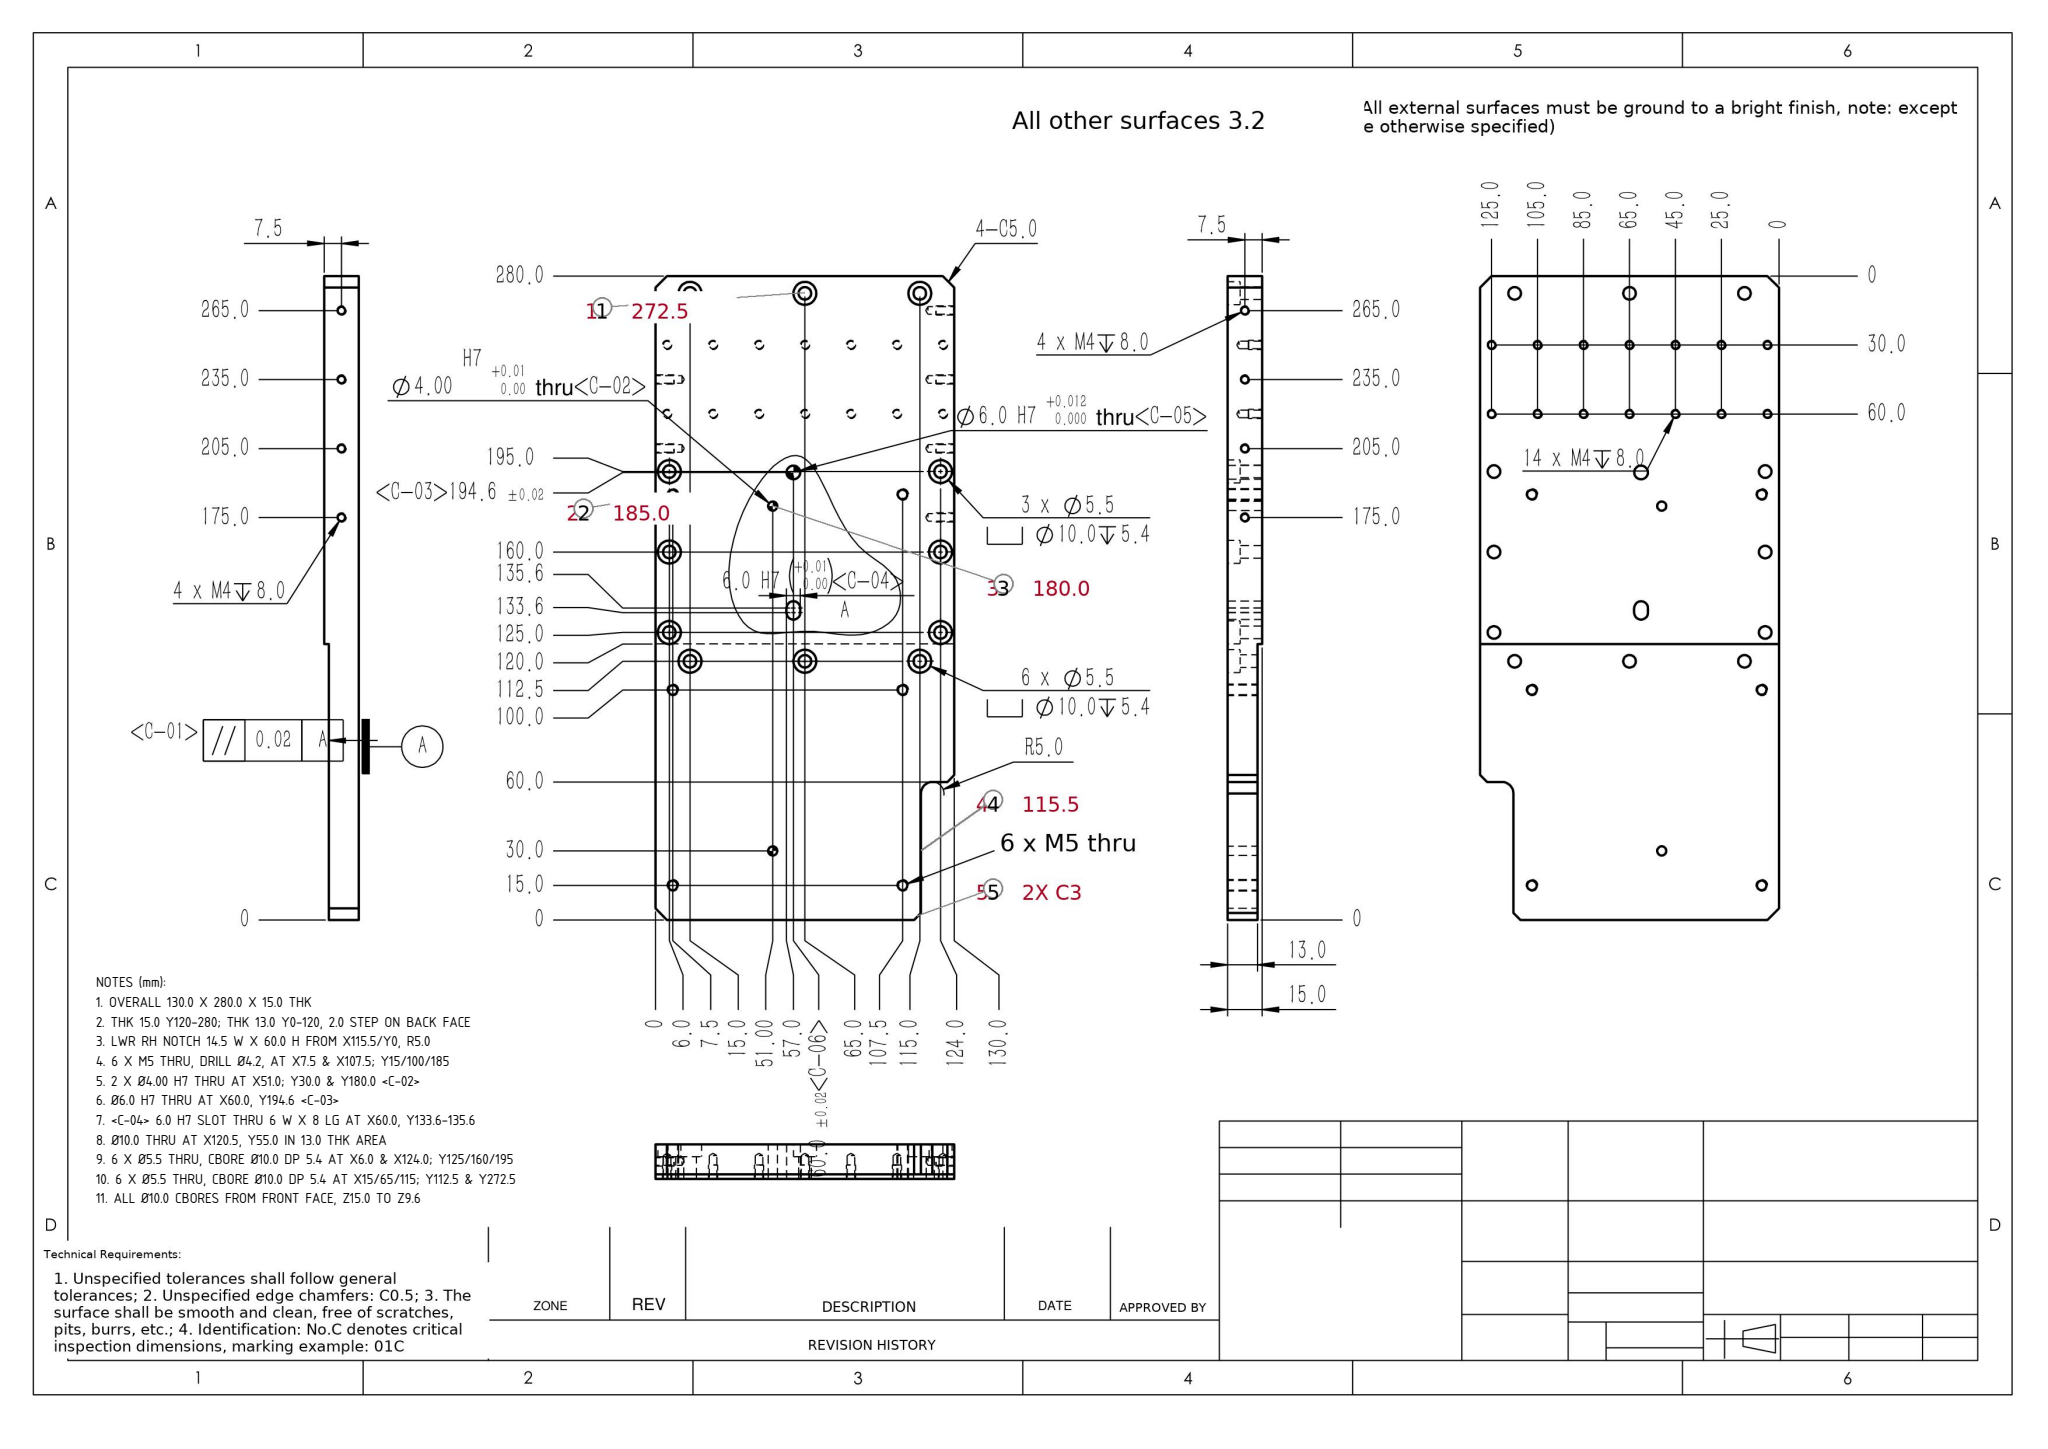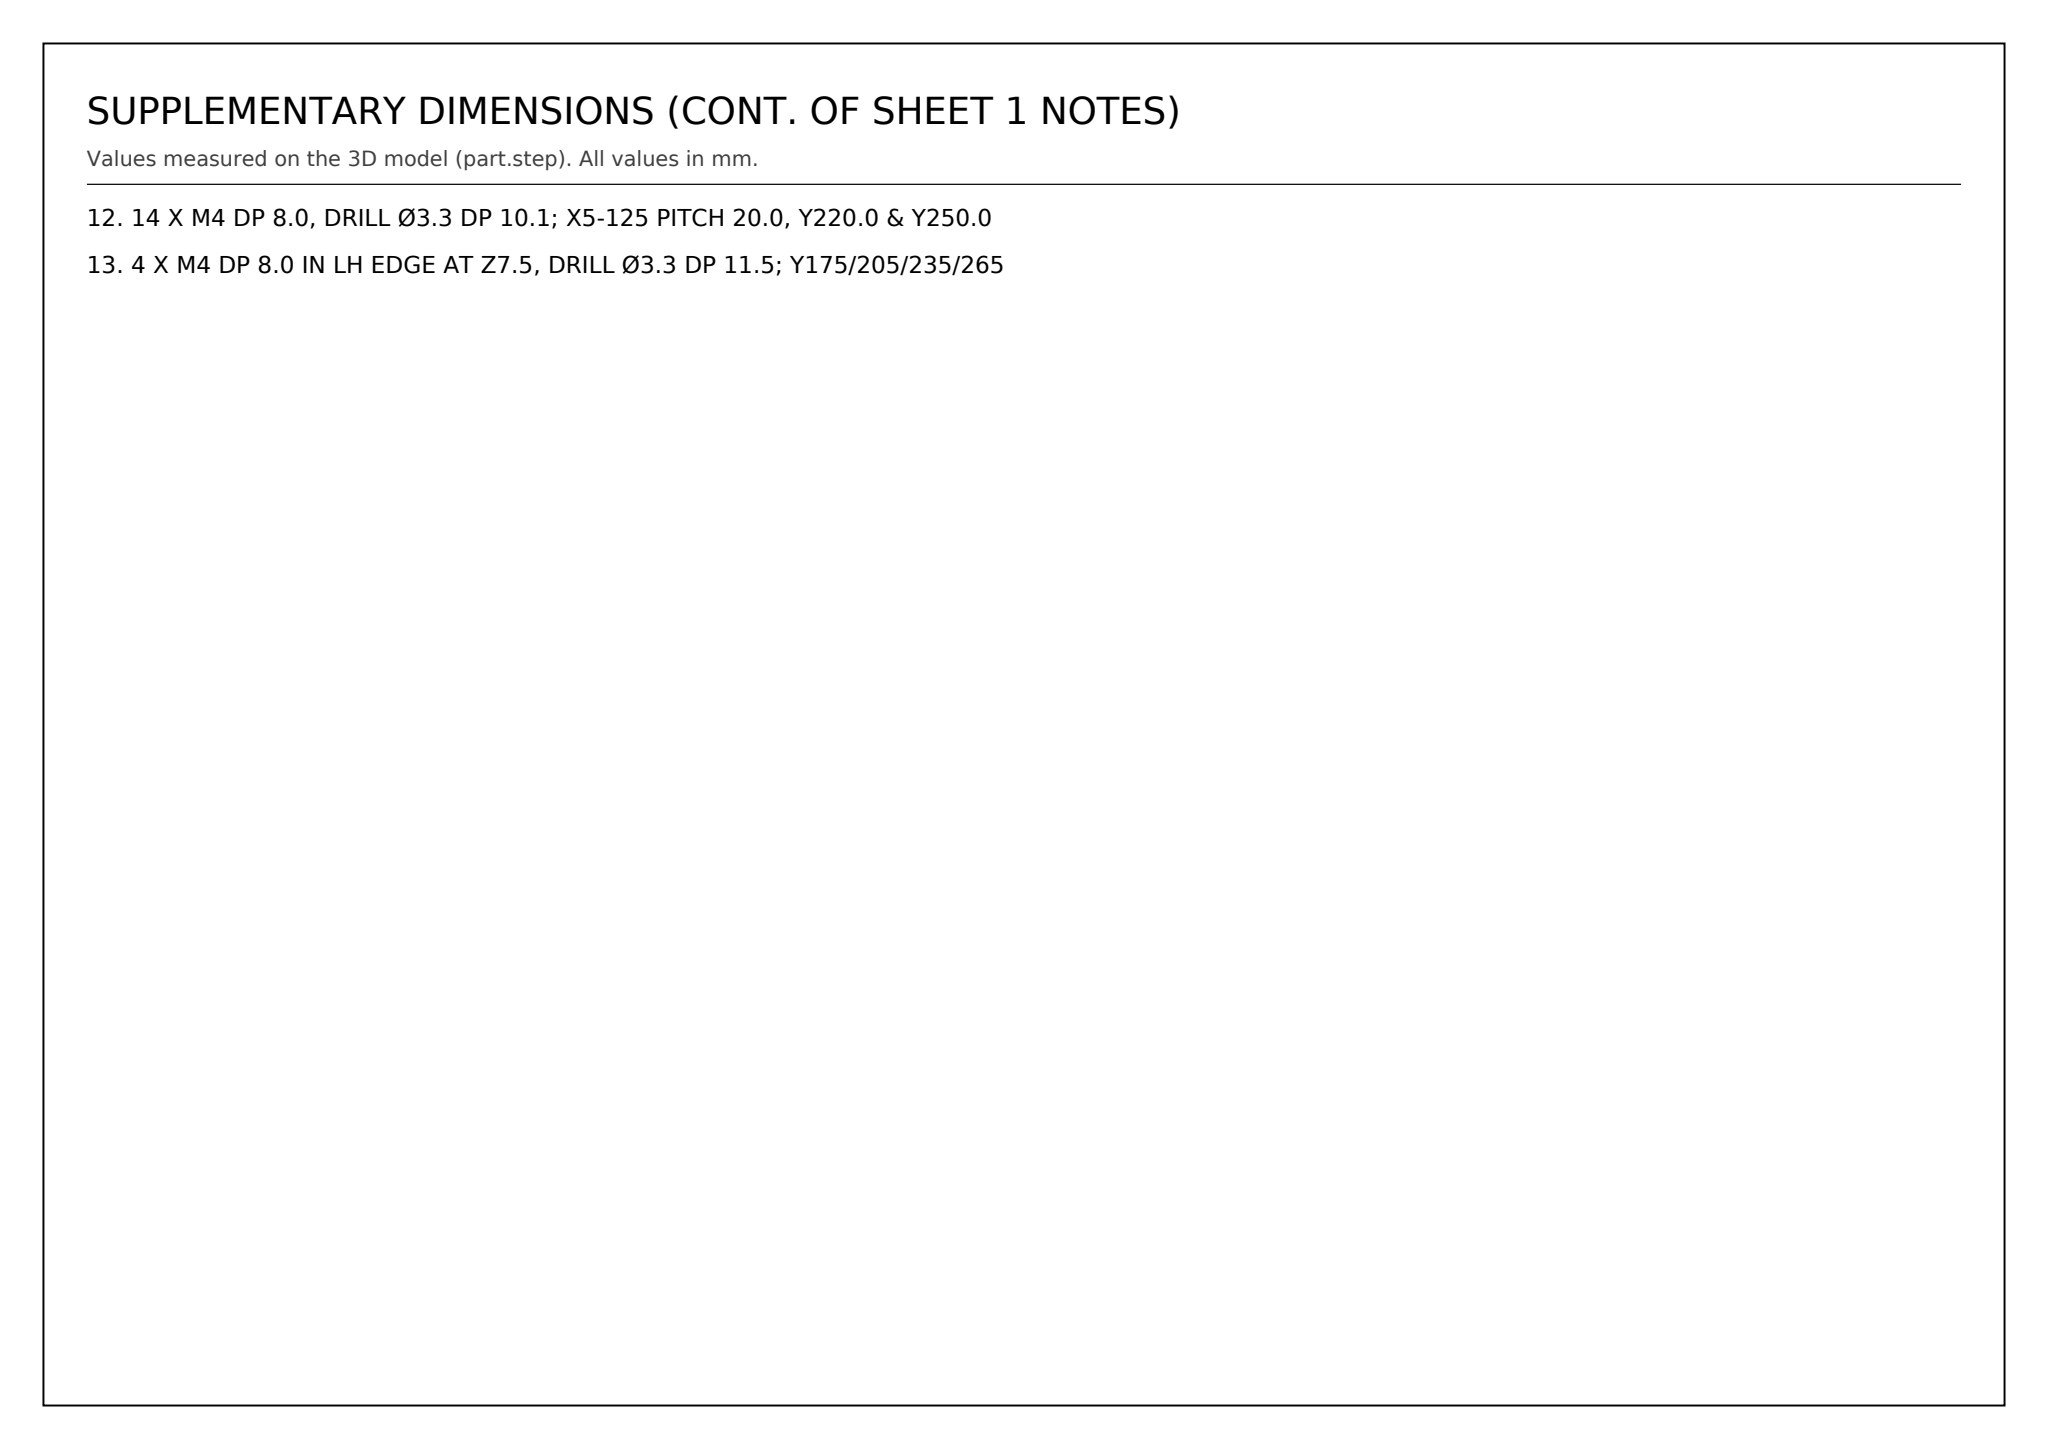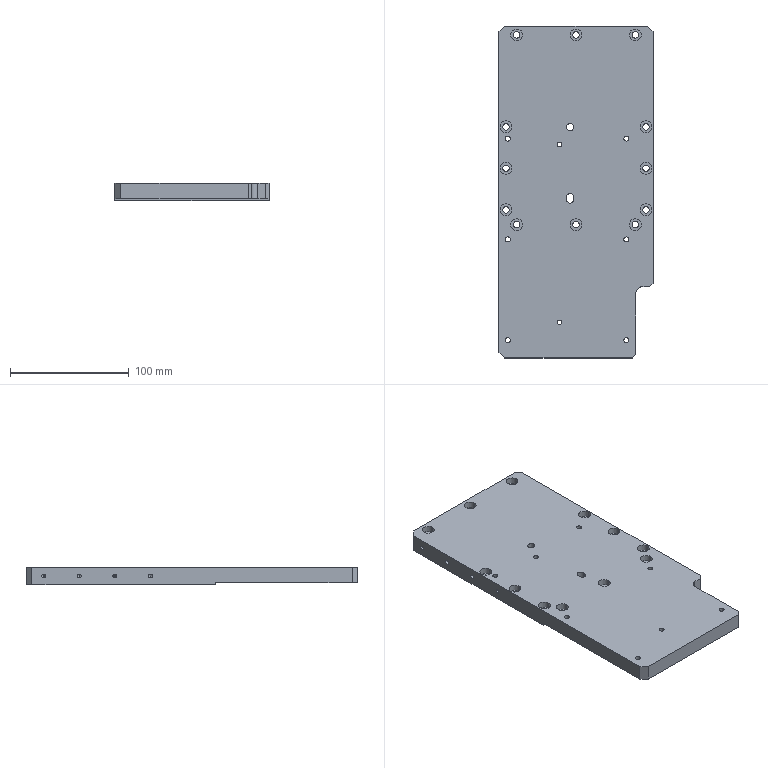Part | SolidWorks | mm | 1 solid | 186 faces | box 130 x 280 x 15 mm | volume 490647 mm3 | cylinder 113 | cone 44 | plane 29 | commonest cylinder face diameters 3.3 x44 10 x25 5.5 x24 4.2 x12 6 x4 4 x4
Drawing notes:
OVERALL 130.0 X 280.0 X 15.0 THK | from the solid: bbox_xyz [130.0, 280.0, 15.0]
THK 15.0 Y120-280; THK 13.0 Y0-120, 2.0 STEP ON BACK FACE | from the solid: z planes 0/2.0/15.0; y plane 120.0; hole len 13.0 at Y15/30/100 vs 15.0 at Y180/185
LWR RH NOTCH 14.5 W X 60.0 H FROM X115.5/Y0, R5.0 | from the solid: x plane 115.5 vs bbox x=130.0; y plane 60.0
6 X M5 THRU, DRILL Ø4.2, AT X7.5 & X107.5; Y15/100/185 | from the solid: Ø4.2 z-holes at (7.5/107.5, 15/100/185), len 13.0 & 15.0 thru
2 X Ø4.00 H7 THRU AT X51.0; Y30.0 & Y180.0 <C-02> | from the solid: Ø4.0 z-holes at (51,30) len 13.0 and (51,180) len 15.0
Ø6.0 H7 THRU AT X60.0, Y194.6 <C-03> | from the solid: Ø6.0 z-hole at (60,194.6) len 15.0
<C-04> 6.0 H7 SLOT THRU 6 W X 8 LG AT X60.0, Y133.6-135.6 | from the solid: Ø6.0 at (60,133.6) & (60,135.6) len 15.0; x planes 57.0 & 63.0
Ø10.0 THRU AT X120.5, Y55.0 IN 13.0 THK AREA | from the solid: Ø10.0 cyl at (120.5,55.0) len 13.0
6 X Ø5.5 THRU, CBORE Ø10.0 DP 5.4 AT X6.0 & X124.0; Y125/160/195 | from the solid: Ø5.5/Ø10.0 at (6,125)(6,160)(6,195)(124,125)(124,160)(124,195)
6 X Ø5.5 THRU, CBORE Ø10.0 DP 5.4 AT X15/65/115; Y112.5 & Y272.5 | from the solid: Ø5.5/Ø10.0 at (15/65/115, 112.5) and (15/65/115, 272.5)
ALL Ø10.0 CBORES FROM FRONT FACE, Z15.0 TO Z9.6 | from the solid: Ø10.0 cyl len 5.4 x12; z plane 9.6 count 12
14 X M4 DP 8.0, DRILL Ø3.3 DP 10.1; X5-125 PITCH 20.0, Y220.0 & Y250.0 | from the solid: Ø3.3 z-axis len 10.1 at x=5,25,45,65,85,105,125; y=220,250
4 X M4 DP 8.0 IN LH EDGE AT Z7.5, DRILL Ø3.3 DP 11.5; Y175/205/235/265 | from the solid: Ø3.3 x-axis len 11.5 at y=175,205,235,265, z=7.5
build123d program:
from build123d import *

# Parameters (mm, degrees)
SKETCH1_W                                       = 130
SKETCH1_H                                       = 280
BOSS_EXTRUDE1_DEPTH                             = 15
SKETCH2_W                                       = 2
SKETCH2_H                                       = 120
CUT_EXTRUDE1_DEPTH                              = 192.638
M5_HEX_SOCKET_HEAD_CAP_SCREW_CBORE2_D           = 5.5
M5_HEX_SOCKET_HEAD_CAP_SCREW_CBORE2_CBORE_D     = 10
M5_HEX_SOCKET_HEAD_CAP_SCREW_CBORE2_CBORE_DEPTH = 5.4
M5_HEX_SOCKET_HEAD_CAP_SCREW_CBORE1_D           = 5.5
M5_HEX_SOCKET_HEAD_CAP_SCREW_CBORE1_CBORE_D     = 10
M5_HEX_SOCKET_HEAD_CAP_SCREW_CBORE1_CBORE_DEPTH = 5.4
M5_TAPPED_HOLE1_D                               = 4.2
SKETCH18_R                                      = 2
CUT_EXTRUDE3_DEPTH                              = 156.081
M5_HEX_SOCKET_HEAD_CAP_SCREW_CBORE3_D           = 5.5
M5_HEX_SOCKET_HEAD_CAP_SCREW_CBORE3_CBORE_D     = 10
M5_HEX_SOCKET_HEAD_CAP_SCREW_CBORE3_CBORE_DEPTH = 5.4
M4_TAPPED_HOLE1_AT_2_COUNT                      = 2
M4_TAPPED_HOLE1_AT_2_PITCH                      = 30
LPATTERN1_COUNT                                 = 4
LPATTERN1_PITCH                                 = 20
LPATTERN2_COUNT                                 = 4
LPATTERN2_PITCH                                 = 30
CHAMFER1_SIZE                                   = 5
SKETCH25_W                                      = 14.5
SKETCH25_H                                      = 60
CUT_EXTRUDE4_DEPTH                              = 156.081
FILLET1_R                                       = 5
CHAMFER2_SIZE                                   = 3
SKETCH26_R                                      = 3
CUT_EXTRUDE5_DEPTH                              = 15


with BuildPart() as part:
    # Sketch1 → Boss-Extrude1 (new body)
    with BuildSketch(Plane.XY):
        Rectangle(SKETCH1_W, SKETCH1_H)
    extrude(amount=BOSS_EXTRUDE1_DEPTH)

    # Sketch2 → Cut-Extrude1 (cut, through all)
    with BuildSketch(Plane.ZY.offset(65)):
        with Locations((1, -80)):
            Rectangle(SKETCH2_W, SKETCH2_H)
    extrude(amount=-CUT_EXTRUDE1_DEPTH, mode=Mode.SUBTRACT)

    # M5 Hex Socket Head Cap Screw CBORE2 (through all)
    with Locations(Plane.XY.offset(15)):
        with Locations((-50, -27.5), (0, -27.5), (50, -27.5)):
            CounterBoreHole(M5_HEX_SOCKET_HEAD_CAP_SCREW_CBORE2_D / 2, M5_HEX_SOCKET_HEAD_CAP_SCREW_CBORE2_CBORE_D / 2, M5_HEX_SOCKET_HEAD_CAP_SCREW_CBORE2_CBORE_DEPTH)

    # M5 Hex Socket Head Cap Screw CBORE1 (through all)
    with Locations(Plane.XY.offset(15)):
        with Locations((-59, 55), (-59, 20), (-59, -15)):
            m5_hex_socket_head_cap_screw_cbore1 = CounterBoreHole(M5_HEX_SOCKET_HEAD_CAP_SCREW_CBORE1_D / 2, M5_HEX_SOCKET_HEAD_CAP_SCREW_CBORE1_CBORE_D / 2, M5_HEX_SOCKET_HEAD_CAP_SCREW_CBORE1_CBORE_DEPTH)

    # Mirror2: M5 Hex Socket Head Cap Screw CBORE1 across plane
    add(m5_hex_socket_head_cap_screw_cbore1.mirror(Plane(origin=(0, 0, 0), x_dir=(0, 0, 1), z_dir=(1, 0, 0))), mode=Mode.SUBTRACT)

    # M5 Tapped Hole1 (through all)
    with Locations(Plane.XY.offset(15)):
        with Locations((-57.5, 45), (-57.5, -40), (-57.5, -125), (42.5, -125), (42.5, -40), (42.5, 45)):
            Hole(M5_TAPPED_HOLE1_D / 2)

    # Sketch18 → Cut-Extrude3 (cut, through all)
    with BuildSketch(Plane.XY.offset(15)):
        with Locations((-14, 40)):
            Circle(SKETCH18_R)
        with Locations((-14, -110)):
            Circle(SKETCH18_R)
    extrude(amount=-CUT_EXTRUDE3_DEPTH, mode=Mode.SUBTRACT)

    # M5 Hex Socket Head Cap Screw CBORE3 (through all)
    with Locations(Plane.XY.offset(15)):
        with Locations((-50, 132.5), (0, 132.5), (50, 132.5)):
            CounterBoreHole(M5_HEX_SOCKET_HEAD_CAP_SCREW_CBORE3_D / 2, M5_HEX_SOCKET_HEAD_CAP_SCREW_CBORE3_CBORE_D / 2, M5_HEX_SOCKET_HEAD_CAP_SCREW_CBORE3_CBORE_DEPTH)

    # Sketch21 → M4 Tapped Hole1 (revolve, cut)
    with BuildSketch(Plane(origin=(0, 110, 0), x_dir=(0, 1, 0), z_dir=(1, 0, 0))):
        Polygon((0, 0), (0, 11.091), (1.65, 10.1), (1.65, 0), align=None)
    m4_tapped_hole1 = revolve(axis=Axis((0, 110, -6.35), (0, 0, 1)), mode=Mode.SUBTRACT)

    # M4 Tapped Hole1 at 2: M4 Tapped Hole1 ×2
    with Locations(*[(0, -i * M4_TAPPED_HOLE1_AT_2_PITCH, 0) for i in range(1, M4_TAPPED_HOLE1_AT_2_COUNT)]):
        add(m4_tapped_hole1, mode=Mode.SUBTRACT)

    # LPattern1: M4 Tapped Hole1 ×4
    with Locations(*[(i * LPATTERN1_PITCH, 0, 0) for i in range(1, LPATTERN1_COUNT)]):
        add(m4_tapped_hole1, mode=Mode.SUBTRACT)

    # LPattern1 copy 1 sketch → LPattern1 copy 1 (revolve, cut)
    with BuildSketch(Plane(origin=(20, 80, 0), x_dir=(0, 1, 0), z_dir=(1, 0, 0))):
        Polygon((0, 0), (0, 11.091), (1.65, 10.1), (1.65, 0), align=None)
    revolve(axis=Axis((20, 80, -6.35), (0, 0, 1)), mode=Mode.SUBTRACT)

    # LPattern1 copy 2 sketch → LPattern1 copy 2 (revolve, cut)
    with BuildSketch(Plane(origin=(40, 80, 0), x_dir=(0, 1, 0), z_dir=(1, 0, 0))):
        Polygon((0, 0), (0, 11.091), (1.65, 10.1), (1.65, 0), align=None)
    revolve(axis=Axis((40, 80, -6.35), (0, 0, 1)), mode=Mode.SUBTRACT)

    # LPattern1 copy 3 sketch → LPattern1 copy 3 (revolve, cut)
    with BuildSketch(Plane(origin=(60, 80, 0), x_dir=(0, 1, 0), z_dir=(1, 0, 0))):
        Polygon((0, 0), (0, 11.091), (1.65, 10.1), (1.65, 0), align=None)
    revolve(axis=Axis((60, 80, -6.35), (0, 0, 1)), mode=Mode.SUBTRACT)

    # Mirror3 copy 1 sketch → Mirror3 copy 1 (revolve, cut)
    with BuildSketch(Plane(origin=(-20, 110, 0), x_dir=(0, 1, 0), z_dir=(-1, 0, 0))):
        Polygon((0, 0), (0, -11.091), (1.65, -10.1), (1.65, 0), align=None)
    revolve(axis=Axis((-20, 110, -6.35), (0, 0, -1)), mode=Mode.SUBTRACT)

    # Mirror3 copy 2 sketch → Mirror3 copy 2 (revolve, cut)
    with BuildSketch(Plane(origin=(-40, 110, 0), x_dir=(0, 1, 0), z_dir=(-1, 0, 0))):
        Polygon((0, 0), (0, -11.091), (1.65, -10.1), (1.65, 0), align=None)
    revolve(axis=Axis((-40, 110, -6.35), (0, 0, -1)), mode=Mode.SUBTRACT)

    # Mirror3 copy 3 sketch → Mirror3 copy 3 (revolve, cut)
    with BuildSketch(Plane(origin=(-60, 110, 0), x_dir=(0, 1, 0), z_dir=(-1, 0, 0))):
        Polygon((0, 0), (0, -11.091), (1.65, -10.1), (1.65, 0), align=None)
    revolve(axis=Axis((-60, 110, -6.35), (0, 0, -1)), mode=Mode.SUBTRACT)

    # Mirror3 copy 4 sketch → Mirror3 copy 4 (revolve, cut)
    with BuildSketch(Plane(origin=(-20, 80, 0), x_dir=(0, 1, 0), z_dir=(-1, 0, 0))):
        Polygon((0, 0), (0, -11.091), (1.65, -10.1), (1.65, 0), align=None)
    revolve(axis=Axis((-20, 80, -6.35), (0, 0, -1)), mode=Mode.SUBTRACT)

    # Mirror3 copy 5 sketch → Mirror3 copy 5 (revolve, cut)
    with BuildSketch(Plane(origin=(-40, 80, 0), x_dir=(0, 1, 0), z_dir=(-1, 0, 0))):
        Polygon((0, 0), (0, -11.091), (1.65, -10.1), (1.65, 0), align=None)
    revolve(axis=Axis((-40, 80, -6.35), (0, 0, -1)), mode=Mode.SUBTRACT)

    # Mirror3 copy 6 sketch → Mirror3 copy 6 (revolve, cut)
    with BuildSketch(Plane(origin=(-60, 80, 0), x_dir=(0, 1, 0), z_dir=(-1, 0, 0))):
        Polygon((0, 0), (0, -11.091), (1.65, -10.1), (1.65, 0), align=None)
    revolve(axis=Axis((-60, 80, -6.35), (0, 0, -1)), mode=Mode.SUBTRACT)

    # Mirror3 copy 7 sketch → Mirror3 copy 7 (revolve, cut)
    with BuildSketch(Plane(origin=(0, 110, 0), x_dir=(0, 1, 0), z_dir=(-1, 0, 0))):
        Polygon((0, 0), (0, -11.091), (1.65, -10.1), (1.65, 0), align=None)
    revolve(axis=Axis((0, 110, -6.35), (0, 0, -1)), mode=Mode.SUBTRACT)

    # Mirror3 copy 8 sketch → Mirror3 copy 8 (revolve, cut)
    with BuildSketch(Plane(origin=(0, 80, 0), x_dir=(0, 1, 0), z_dir=(-1, 0, 0))):
        Polygon((0, 0), (0, -11.091), (1.65, -10.1), (1.65, 0), align=None)
    revolve(axis=Axis((0, 80, -6.35), (0, 0, -1)), mode=Mode.SUBTRACT)

    # Sketch23 → M4 Tapped Hole2 (revolve, cut)
    with BuildSketch(Plane(origin=(65, 125, 7.5), x_dir=(0, 0, -1), z_dir=(0, 1, 0))):
        Polygon((0, 0), (0, 12.491), (1.65, 11.5), (1.65, 0), align=None)
    m4_tapped_hole2 = revolve(axis=Axis((71.35, 125, 7.5), (-1, 0, 0)), mode=Mode.SUBTRACT)

    # LPattern2: M4 Tapped Hole2 ×4
    with Locations(*[(0, -i * LPATTERN2_PITCH, 0) for i in range(1, LPATTERN2_COUNT)]):
        add(m4_tapped_hole2, mode=Mode.SUBTRACT)

    # Mirror4: M4 Tapped Hole2 across plane
    add(m4_tapped_hole2.mirror(Plane(origin=(0, 0, 0), x_dir=(0, 0, 1), z_dir=(1, 0, 0))), mode=Mode.SUBTRACT)

    # Mirror4 copy 1 sketch → Mirror4 copy 1 (revolve, cut)
    with BuildSketch(Plane(origin=(-65, 95, 7.5), x_dir=(0, 0, -1), z_dir=(0, 1, 0))):
        Polygon((0, 0), (0, -12.491), (1.65, -11.5), (1.65, 0), align=None)
    revolve(axis=Axis((-71.35, 95, 7.5), (-1, 0, 0)), mode=Mode.SUBTRACT)

    # Mirror4 copy 2 sketch → Mirror4 copy 2 (revolve, cut)
    with BuildSketch(Plane(origin=(-65, 65, 7.5), x_dir=(0, 0, -1), z_dir=(0, 1, 0))):
        Polygon((0, 0), (0, -12.491), (1.65, -11.5), (1.65, 0), align=None)
    revolve(axis=Axis((-71.35, 65, 7.5), (-1, 0, 0)), mode=Mode.SUBTRACT)

    # Mirror4 copy 3 sketch → Mirror4 copy 3 (revolve, cut)
    with BuildSketch(Plane(origin=(-65, 35, 7.5), x_dir=(0, 0, -1), z_dir=(0, 1, 0))):
        Polygon((0, 0), (0, -12.491), (1.65, -11.5), (1.65, 0), align=None)
    revolve(axis=Axis((-71.35, 35, 7.5), (-1, 0, 0)), mode=Mode.SUBTRACT)

    # Chamfer1
    chamfer1_edges = [part.edges().sort_by_distance(p)[0] for p in [
        (65, -140, 8.5),
        (-65, -140, 8.5),
        (-65, 140, 7.5),
        (65, 140, 7.5),
    ]]
    chamfer(chamfer1_edges, length=CHAMFER1_SIZE)

    # Sketch25 → Cut-Extrude4 (cut, through all)
    with BuildSketch(Plane.XY.offset(15)):
        with Locations((57.75, -110)):
            Rectangle(SKETCH25_W, SKETCH25_H)
    extrude(amount=-CUT_EXTRUDE4_DEPTH, mode=Mode.SUBTRACT)

    # Fillet1
    fillet1_edges = [part.edges().sort_by_distance(p)[0] for p in [
        (50.5, -80, 8.5),
    ]]
    fillet(fillet1_edges, radius=FILLET1_R)

    # Chamfer2
    chamfer2_edges = [part.edges().sort_by_distance(p)[0] for p in [
        (50.5, -140, 8.5),
        (65, -80, 8.5),
    ]]
    chamfer(chamfer2_edges, length=CHAMFER2_SIZE)

    # Sketch26 → Cut-Extrude5 (cut)
    with BuildSketch(Plane.XY.offset(15)):
        with Locations((-5, 54.6)):
            Circle(SKETCH26_R)
        with BuildLine():
            Line((-8, -6.4), (-8, -4.4))
            ThreePointArc((-8, -4.4), (-5, -1.4), (-2, -4.4))
            Line((-2, -4.4), (-2, -6.4))
            ThreePointArc((-2, -6.4), (-5, -9.4), (-8, -6.4))
        make_face()
    extrude(amount=-CUT_EXTRUDE5_DEPTH, mode=Mode.SUBTRACT)


solid = part.part